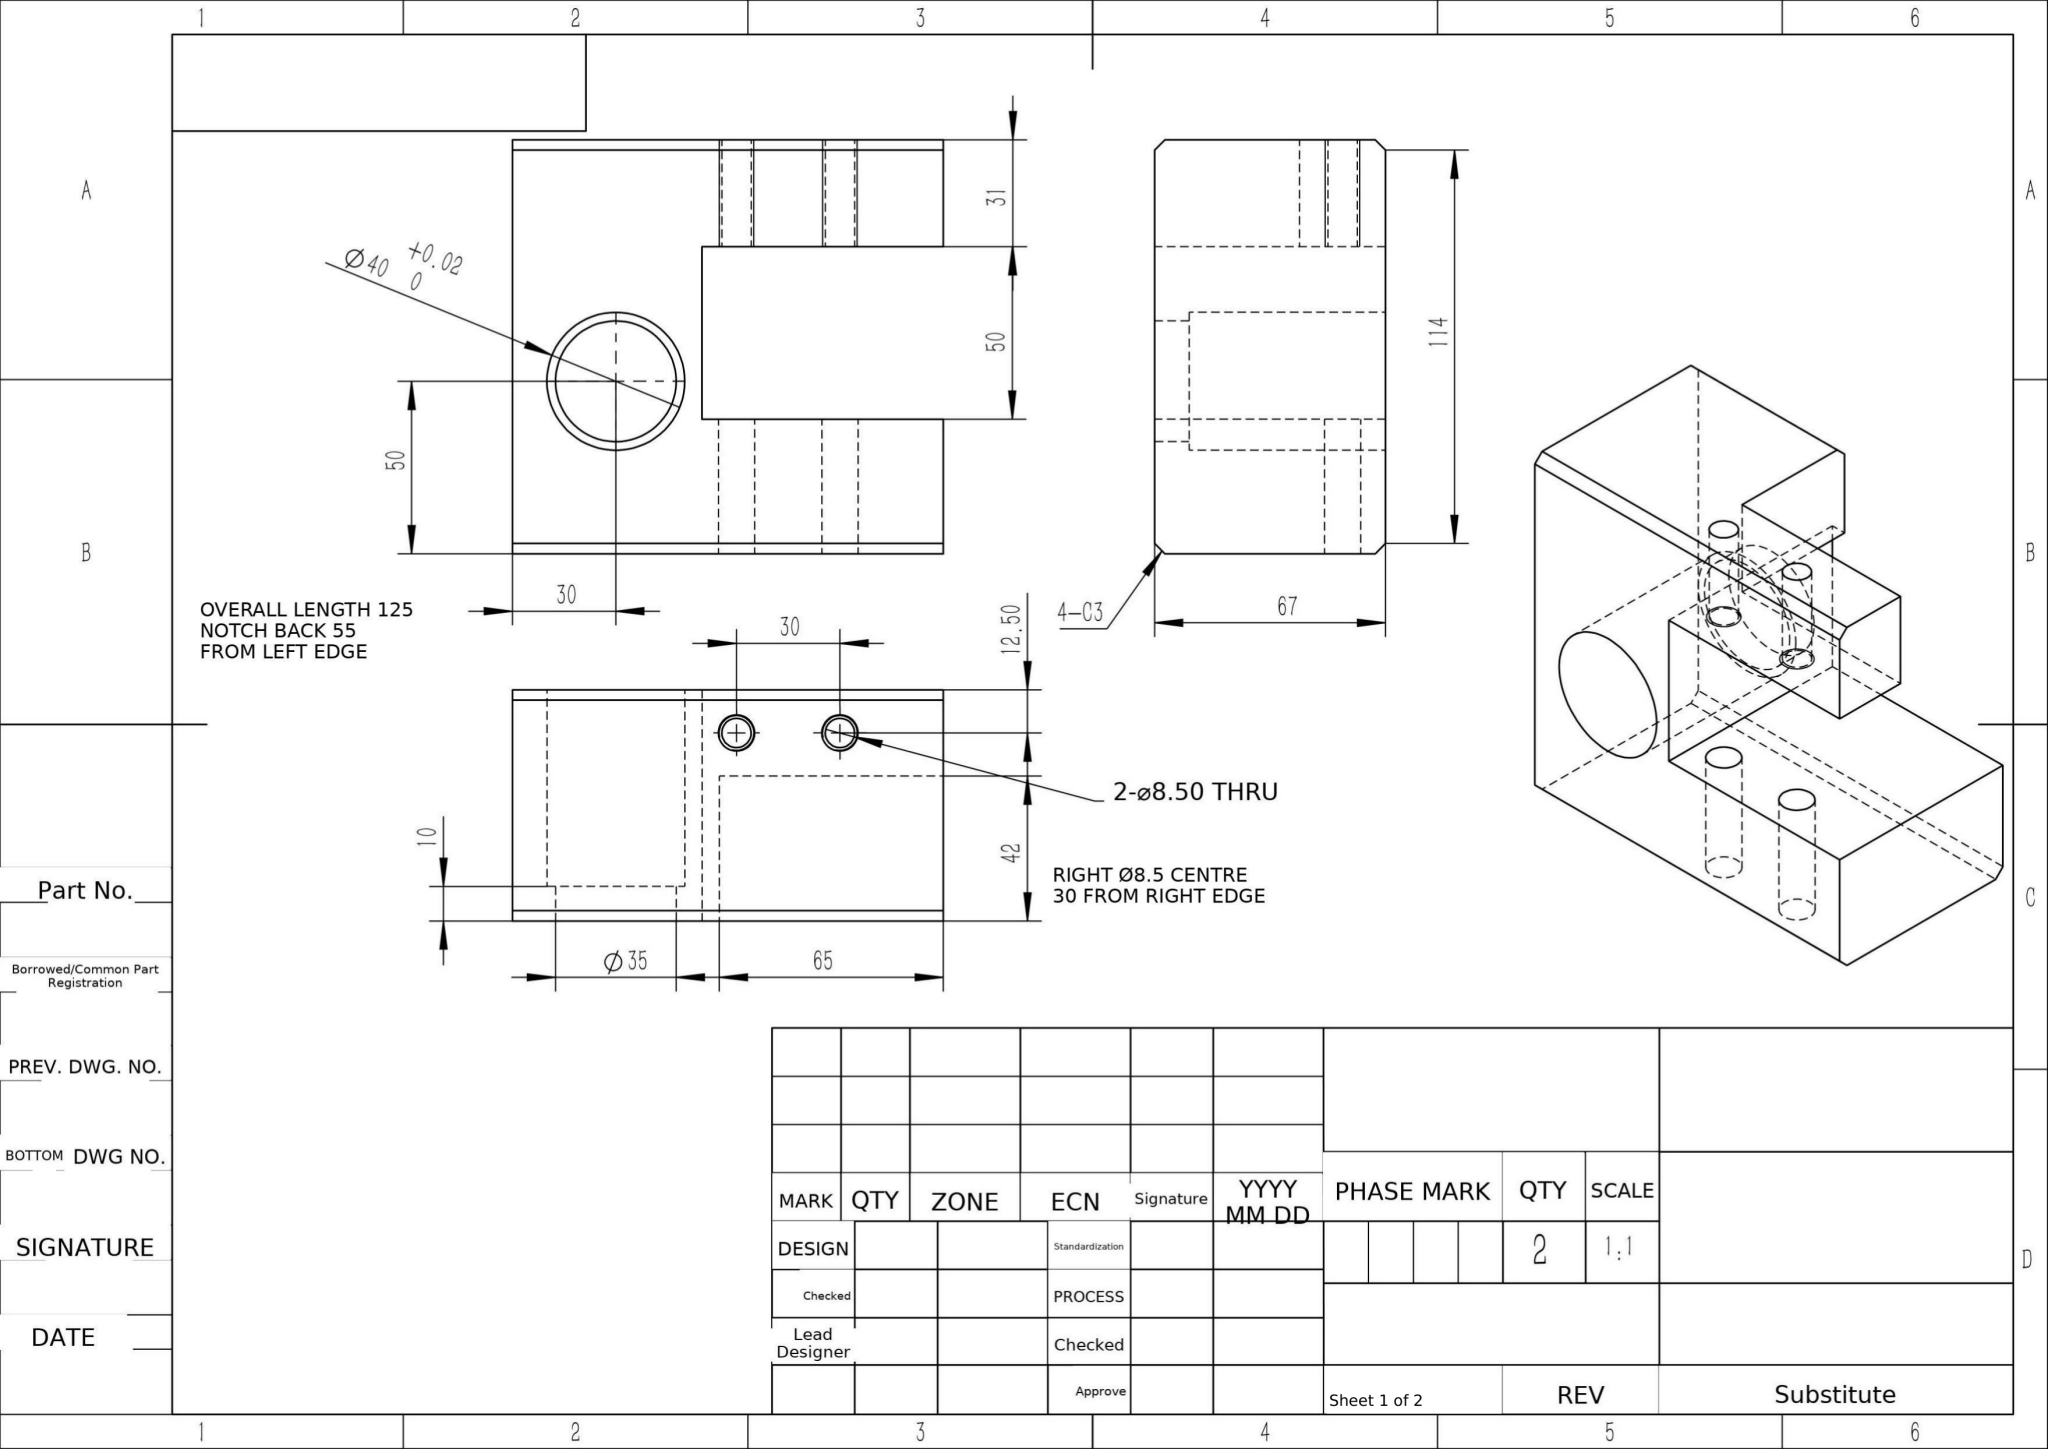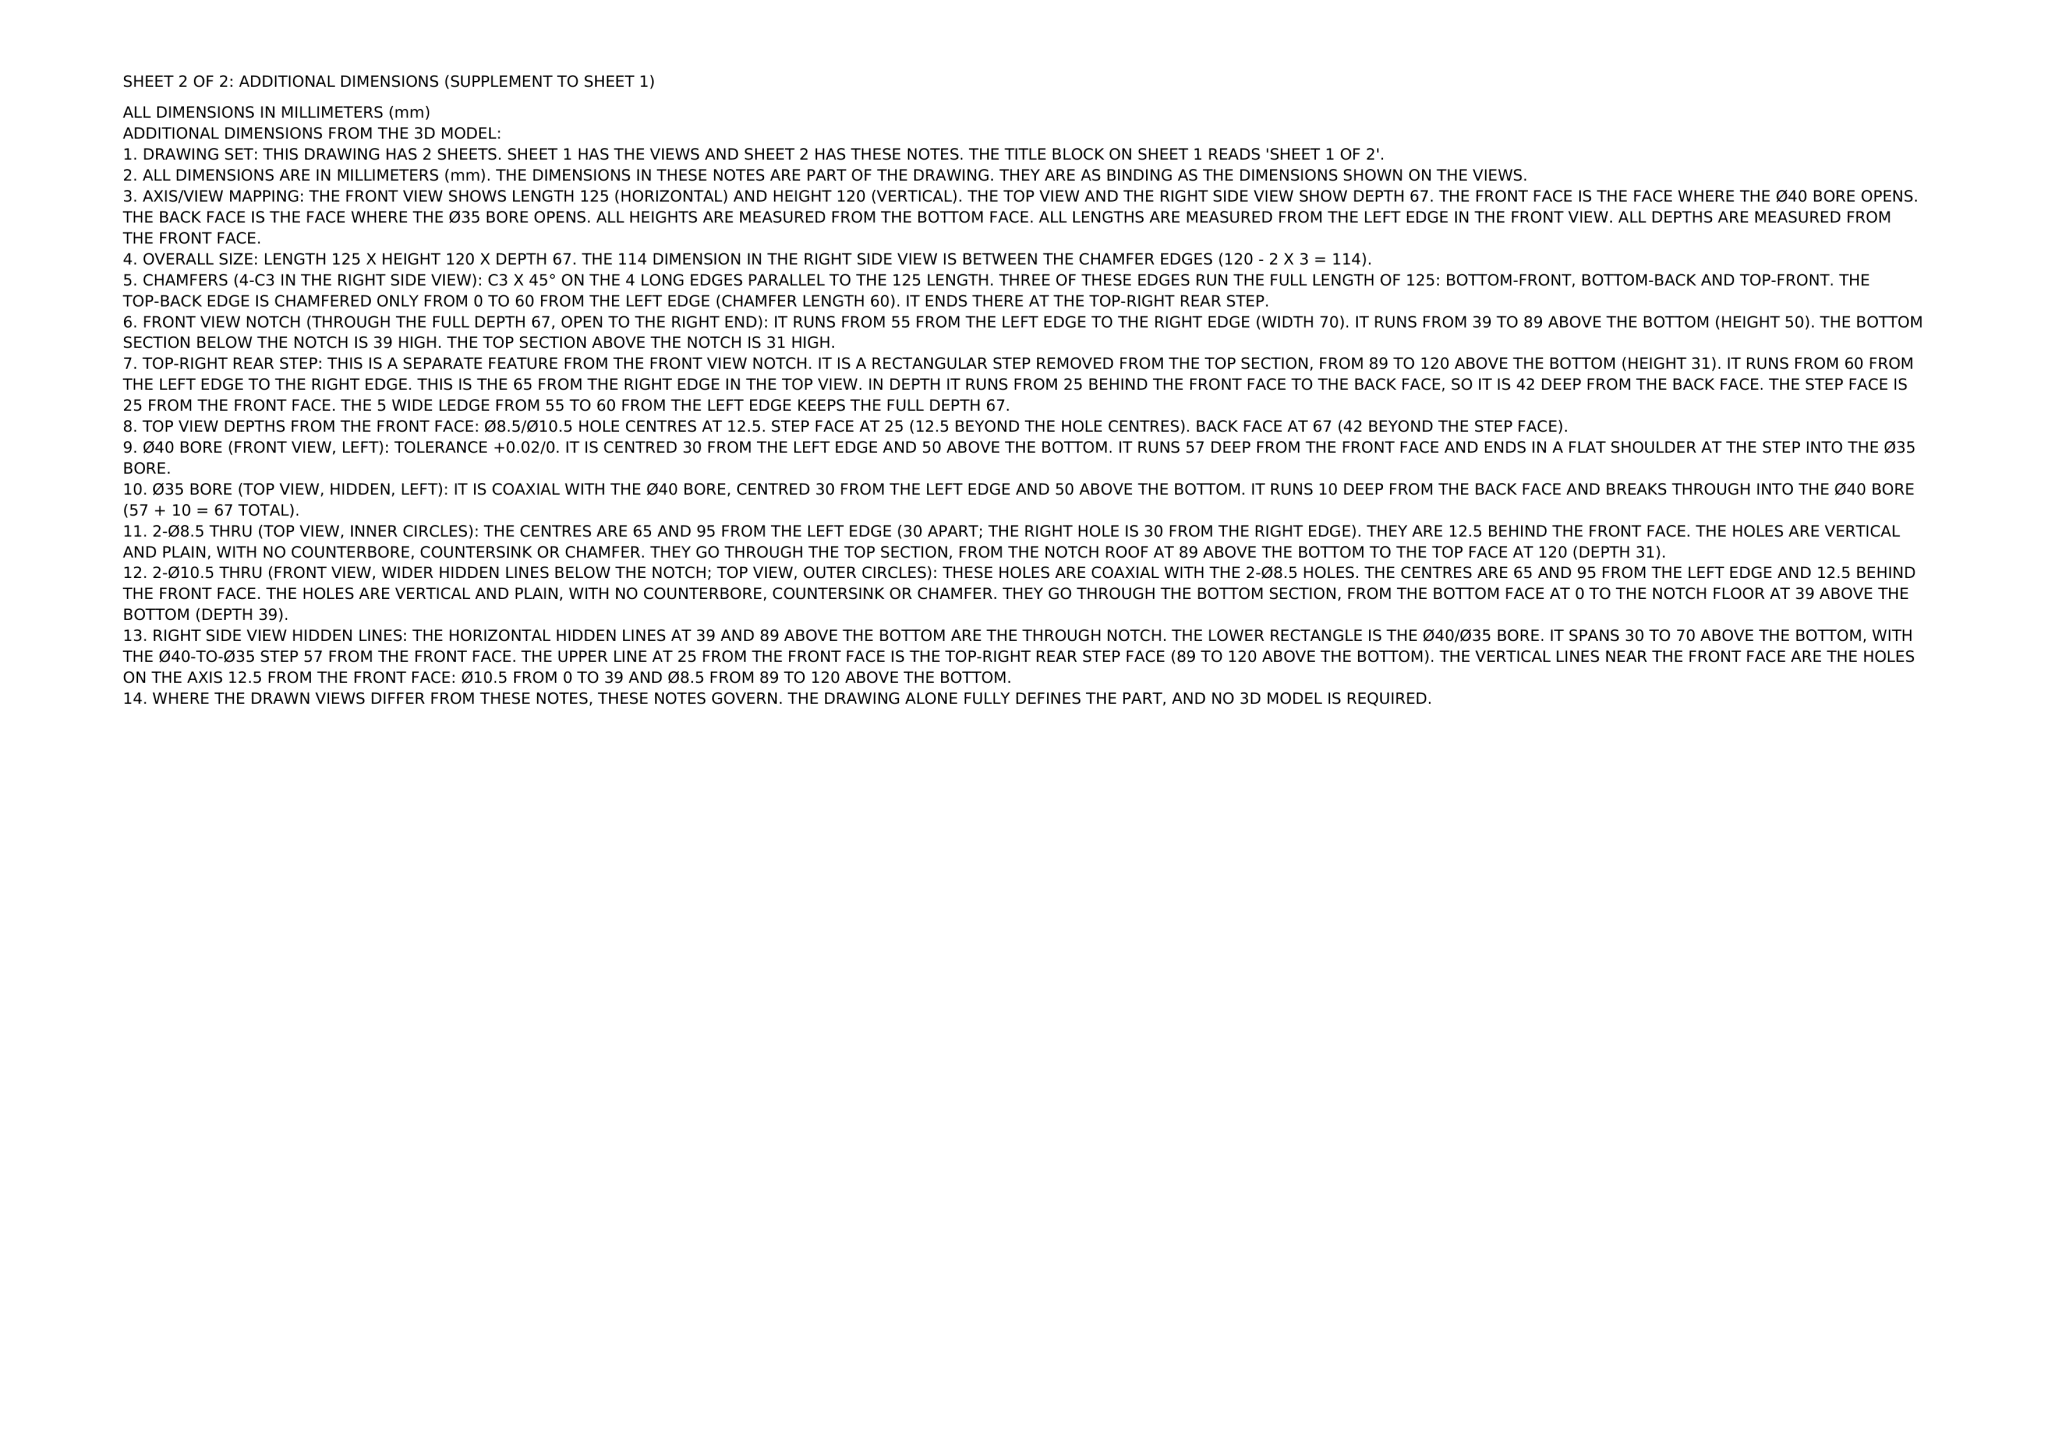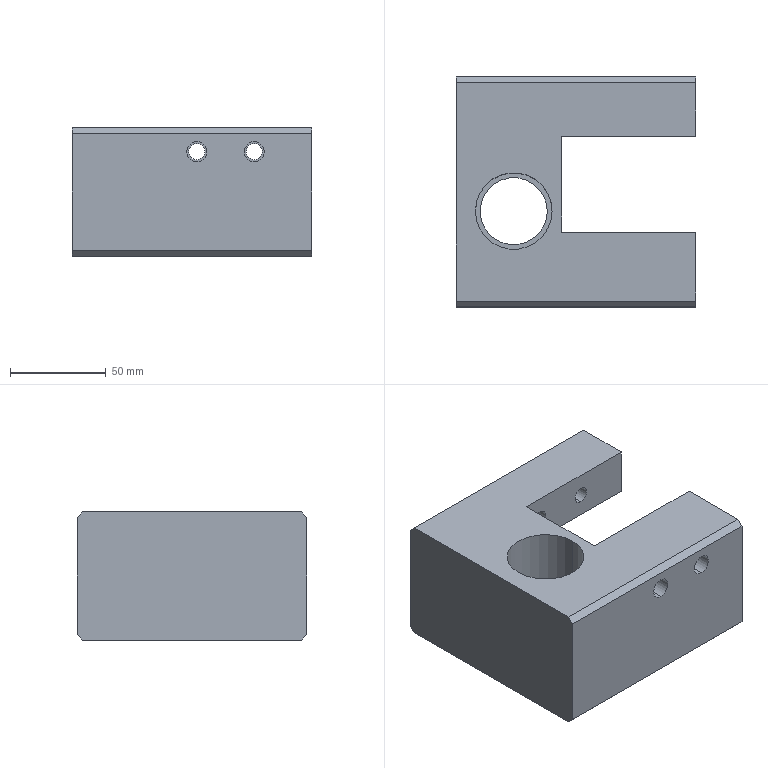Part | NX | mm | C-Shaped Guide Block | 1 solid | 29 faces | box 125 x 120 x 67 mm | volume 592391 mm3 | plane 17 | cylinder 12 | commonest cylinder face diameters 10.5 x4 8.5 x4 40 x2 35 x2